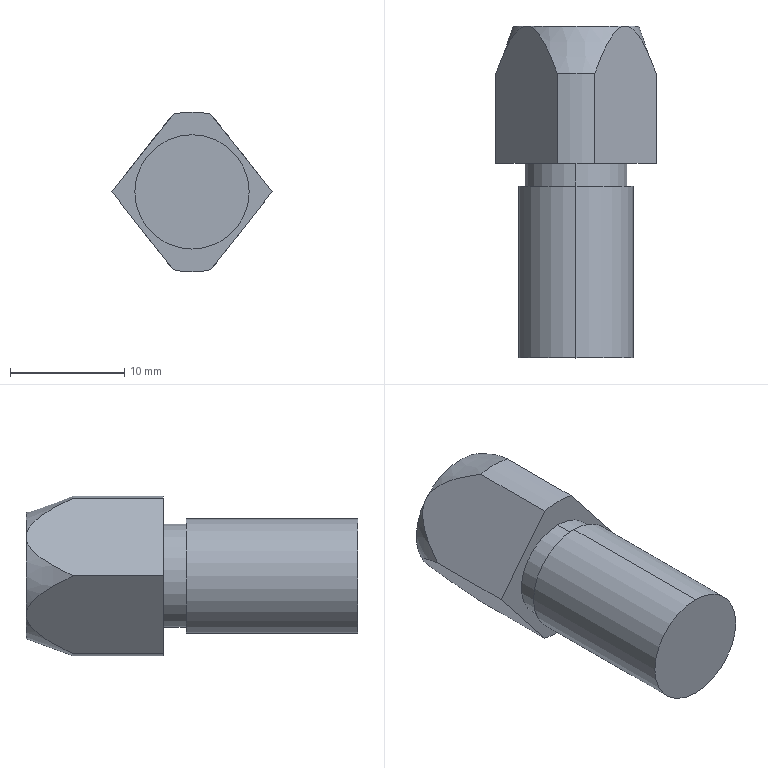Component | SolidWorks | 10-14DiamondPin-1 | 1 solid | 20 faces | box 14 x 29 x 14 mm | volume 2690 mm3 | plane 8 | cylinder 7 | cone 5 | commonest cylinder face diameters 14 x3 9 x2 10 x2
STEP:
#1=COLOUR_RGB('',0.7922,0.8196,0.9333);
#2=FILL_AREA_STYLE_COLOUR('',#1);
#3=FILL_AREA_STYLE('',(#2));
#4=SURFACE_STYLE_FILL_AREA(#3);
#5=SURFACE_SIDE_STYLE('',(#4));
#6=SURFACE_STYLE_USAGE(.BOTH.,#5);
#7=PRESENTATION_STYLE_ASSIGNMENT((#6));
#8=CARTESIAN_POINT('',(2.495,3.663,1.87));
#9=VERTEX_POINT('',#8);
#10=CARTESIAN_POINT('',(2.495,3.663,2.224));
#11=VERTEX_POINT('',#10);
#12=CARTESIAN_POINT('',(2.495,3.663,2.047));
#13=DIRECTION('',(0.,-1.,0.));
#14=DIRECTION('',(0.,0.,-1.));
#15=AXIS2_PLACEMENT_3D('',#12,#13,#14);
#16=CIRCLE('',#15,0.1772);
#17=EDGE_CURVE('',#9,#11,#16,.T.);
#18=ORIENTED_EDGE('',*,*,#17,.T.);
#19=CARTESIAN_POINT('',(2.495,3.585,2.224));
#20=VERTEX_POINT('',#19);
#21=CARTESIAN_POINT('',(2.495,2.994,2.224));
#22=DIRECTION('',(0.,-1.,0.));
#23=VECTOR('',#22,39.37);
#24=LINE('',#21,#23);
#25=EDGE_CURVE('',#11,#20,#24,.T.);
#26=ORIENTED_EDGE('',*,*,#25,.T.);
#27=CARTESIAN_POINT('',(2.495,3.585,1.87));
#28=VERTEX_POINT('',#27);
#29=CARTESIAN_POINT('',(2.495,3.585,2.047));
#30=DIRECTION('',(0.,-1.,0.));
#31=DIRECTION('',(0.,0.,-1.));
#32=AXIS2_PLACEMENT_3D('',#29,#30,#31);
#33=CIRCLE('',#32,0.1772);
#34=EDGE_CURVE('',#28,#20,#33,.T.);
#35=ORIENTED_EDGE('',*,*,#34,.F.);
#36=CARTESIAN_POINT('',(2.495,2.994,1.87));
#37=DIRECTION('',(0.,-1.,0.));
#38=VECTOR('',#37,39.37);
#39=LINE('',#36,#38);
#40=EDGE_CURVE('',#9,#28,#39,.T.);
#41=ORIENTED_EDGE('',*,*,#40,.F.);
#42=EDGE_LOOP('',(#18,#26,#35,#41));
#43=FACE_OUTER_BOUND('',#42,.T.);
#44=CARTESIAN_POINT('',(2.495,2.994,2.047));
#45=DIRECTION('',(0.,-1.,0.));
#46=DIRECTION('',(0.,0.,-1.));
#47=AXIS2_PLACEMENT_3D('',#44,#45,#46);
#48=CYLINDRICAL_SURFACE('',#47,0.1772);
#49=ADVANCED_FACE('',(#43),#48,.T.);
#50=CARTESIAN_POINT('',(2.495,3.585,1.85));
#51=VERTEX_POINT('',#50);
#52=CARTESIAN_POINT('',(2.495,3.585,2.244));
#53=VERTEX_POINT('',#52);
#54=CARTESIAN_POINT('',(2.495,3.585,2.047));
#55=DIRECTION('',(0.,-1.,0.));
#56=DIRECTION('',(0.,0.,-1.));
#57=AXIS2_PLACEMENT_3D('',#54,#55,#56);
#58=CIRCLE('',#57,0.1969);
#59=EDGE_CURVE('',#51,#53,#58,.T.);
#60=ORIENTED_EDGE('',*,*,#59,.T.);
#61=CARTESIAN_POINT('',(2.495,2.994,2.244));
#62=VERTEX_POINT('',#61);
#63=CARTESIAN_POINT('',(2.495,2.994,2.244));
#64=DIRECTION('',(0.,-1.,0.));
#65=VECTOR('',#64,39.37);
#66=LINE('',#63,#65);
#67=EDGE_CURVE('',#53,#62,#66,.T.);
#68=ORIENTED_EDGE('',*,*,#67,.T.);
#69=CARTESIAN_POINT('',(2.495,2.994,1.85));
#70=VERTEX_POINT('',#69);
#71=CARTESIAN_POINT('',(2.495,2.994,2.047));
#72=DIRECTION('',(0.,-1.,0.));
#73=DIRECTION('',(0.,0.,-1.));
#74=AXIS2_PLACEMENT_3D('',#71,#72,#73);
#75=CIRCLE('',#74,0.1969);
#76=EDGE_CURVE('',#70,#62,#75,.T.);
#77=ORIENTED_EDGE('',*,*,#76,.F.);
#78=CARTESIAN_POINT('',(2.495,2.994,1.85));
#79=DIRECTION('',(0.,-1.,0.));
#80=VECTOR('',#79,39.37);
#81=LINE('',#78,#80);
#82=EDGE_CURVE('',#51,#70,#81,.T.);
#83=ORIENTED_EDGE('',*,*,#82,.F.);
#84=EDGE_LOOP('',(#60,#68,#77,#83));
#85=FACE_OUTER_BOUND('',#84,.T.);
#86=CARTESIAN_POINT('',(2.495,2.994,2.047));
#87=DIRECTION('',(0.,-1.,0.));
#88=DIRECTION('',(0.,0.,-1.));
#89=AXIS2_PLACEMENT_3D('',#86,#87,#88);
#90=CYLINDRICAL_SURFACE('',#89,0.1969);
#91=ADVANCED_FACE('',(#85),#90,.T.);
#92=CARTESIAN_POINT('',(2.495,4.136,1.831));
#93=VERTEX_POINT('',#92);
#94=CARTESIAN_POINT('',(2.325,4.136,1.913));
#95=VERTEX_POINT('',#94);
#96=CARTESIAN_POINT('',(2.495,4.136,2.047));
#97=DIRECTION('',(0.,1.,0.));
#98=DIRECTION('',(0.,0.,1.));
#99=AXIS2_PLACEMENT_3D('',#96,#97,#98);
#100=CIRCLE('',#99,0.2165);
#101=EDGE_CURVE('',#93,#95,#100,.T.);
#102=ORIENTED_EDGE('',*,*,#101,.F.);
#103=CARTESIAN_POINT('',(2.495,3.973,1.772));
#104=VERTEX_POINT('',#103);
#105=CARTESIAN_POINT('',(2.495,3.973,1.772));
#106=DIRECTION('',(0.,-0.9397,-0.342));
#107=VECTOR('',#106,39.37);
#108=LINE('',#105,#107);
#109=EDGE_CURVE('',#93,#104,#108,.T.);
#110=ORIENTED_EDGE('',*,*,#109,.T.);
#111=CARTESIAN_POINT('',(2.431,3.973,1.779));
#112=VERTEX_POINT('',#111);
#113=CARTESIAN_POINT('',(2.495,3.973,2.047));
#114=DIRECTION('',(0.,-1.,0.));
#115=DIRECTION('',(0.,0.,1.));
#116=AXIS2_PLACEMENT_3D('',#113,#114,#115);
#117=CIRCLE('',#116,0.2756);
#118=EDGE_CURVE('',#112,#104,#117,.T.);
#119=ORIENTED_EDGE('',*,*,#118,.F.);
#120=CARTESIAN_POINT('',(2.325,4.136,1.913));
#121=CARTESIAN_POINT('',(2.328,4.136,1.909));
#122=CARTESIAN_POINT('',(2.331,4.135,1.905));
#123=CARTESIAN_POINT('',(2.338,4.133,1.897));
#124=CARTESIAN_POINT('',(2.341,4.132,1.894));
#125=CARTESIAN_POINT('',(2.35,4.126,1.882));
#126=CARTESIAN_POINT('',(2.355,4.121,1.875));
#127=CARTESIAN_POINT('',(2.366,4.11,1.862));
#128=CARTESIAN_POINT('',(2.37,4.103,1.856));
#129=CARTESIAN_POINT('',(2.379,4.089,1.844));
#130=CARTESIAN_POINT('',(2.384,4.082,1.839));
#131=CARTESIAN_POINT('',(2.396,4.058,1.823));
#132=CARTESIAN_POINT('',(2.404,4.042,1.814));
#133=CARTESIAN_POINT('',(2.418,4.008,1.796));
#134=CARTESIAN_POINT('',(2.424,3.991,1.787));
#135=CARTESIAN_POINT('',(2.431,3.973,1.779));
#136=B_SPLINE_CURVE_WITH_KNOTS('',3,(#120,#121,#122,#123,#124,#125,#126,#127,#128,#129,#130,#131,#132,#133,#134,#135),.UNSPECIFIED.,.F.,.F.,(4,2,2,2,2,2,2,4),(0.006199,0.006588,0.006976,0.007754,0.008531,0.009309,0.01086,0.01242),.UNSPECIFIED.);
#137=EDGE_CURVE('',#95,#112,#136,.T.);
#138=ORIENTED_EDGE('',*,*,#137,.F.);
#139=EDGE_LOOP('',(#102,#110,#119,#138));
#140=FACE_OUTER_BOUND('',#139,.T.);
#141=CARTESIAN_POINT('',(2.495,3.973,2.047));
#142=DIRECTION('',(0.,-1.,0.));
#143=DIRECTION('',(0.,0.,-1.));
#144=AXIS2_PLACEMENT_3D('',#141,#142,#143);
#145=CONICAL_SURFACE('',#144,0.2756,0.3491);
#146=ADVANCED_FACE('',(#140),#145,.T.);
#147=ORIENTED_EDGE('',*,*,#118,.T.);
#148=CARTESIAN_POINT('',(2.495,3.663,1.772));
#149=VERTEX_POINT('',#148);
#150=CARTESIAN_POINT('',(2.495,2.994,1.772));
#151=DIRECTION('',(0.,-1.,0.));
#152=VECTOR('',#151,39.37);
#153=LINE('',#150,#152);
#154=EDGE_CURVE('',#104,#149,#153,.T.);
#155=ORIENTED_EDGE('',*,*,#154,.T.);
#156=CARTESIAN_POINT('',(2.431,3.663,1.779));
#157=VERTEX_POINT('',#156);
#158=CARTESIAN_POINT('',(2.495,3.663,2.047));
#159=DIRECTION('',(0.,-1.,0.));
#160=DIRECTION('',(0.,0.,-1.));
#161=AXIS2_PLACEMENT_3D('',#158,#159,#160);
#162=CIRCLE('',#161,0.2756);
#163=EDGE_CURVE('',#157,#149,#162,.T.);
#164=ORIENTED_EDGE('',*,*,#163,.F.);
#165=CARTESIAN_POINT('',(2.431,3.348,1.779));
#166=DIRECTION('',(0.,1.,0.));
#167=VECTOR('',#166,39.37);
#168=LINE('',#165,#167);
#169=EDGE_CURVE('',#157,#112,#168,.T.);
#170=ORIENTED_EDGE('',*,*,#169,.T.);
#171=EDGE_LOOP('',(#147,#155,#164,#170));
#172=FACE_OUTER_BOUND('',#171,.T.);
#173=CARTESIAN_POINT('',(2.495,2.994,2.047));
#174=DIRECTION('',(0.,-1.,0.));
#175=DIRECTION('',(0.,0.,-1.));
#176=AXIS2_PLACEMENT_3D('',#173,#174,#175);
#177=CYLINDRICAL_SURFACE('',#176,0.2756);
#178=ADVANCED_FACE('',(#172),#177,.T.);
#179=CARTESIAN_POINT('',(2.22,3.973,2.047));
#180=VERTEX_POINT('',#179);
#181=CARTESIAN_POINT('',(2.22,3.973,2.047));
#182=CARTESIAN_POINT('',(2.226,3.991,2.039));
#183=CARTESIAN_POINT('',(2.233,4.008,2.031));
#184=CARTESIAN_POINT('',(2.247,4.042,2.013));
#185=CARTESIAN_POINT('',(2.254,4.058,2.003));
#186=CARTESIAN_POINT('',(2.267,4.082,1.988));
#187=CARTESIAN_POINT('',(2.271,4.089,1.982));
#188=CARTESIAN_POINT('',(2.28,4.103,1.971));
#189=CARTESIAN_POINT('',(2.285,4.11,1.964));
#190=CARTESIAN_POINT('',(2.295,4.121,1.951));
#191=CARTESIAN_POINT('',(2.301,4.126,1.944));
#192=CARTESIAN_POINT('',(2.31,4.132,1.933));
#193=CARTESIAN_POINT('',(2.313,4.133,1.929));
#194=CARTESIAN_POINT('',(2.319,4.135,1.921));
#195=CARTESIAN_POINT('',(2.322,4.136,1.917));
#196=CARTESIAN_POINT('',(2.325,4.136,1.913));
#197=B_SPLINE_CURVE_WITH_KNOTS('',3,(#181,#182,#183,#184,#185,#186,#187,#188,#189,#190,#191,#192,#193,#194,#195,#196),.UNSPECIFIED.,.F.,.F.,(4,2,2,2,2,2,2,4),(0.00000023,0.00155,0.0031,0.003875,0.004649,0.005424,0.005812,0.006199),.UNSPECIFIED.);
#198=EDGE_CURVE('',#180,#95,#197,.T.);
#199=ORIENTED_EDGE('',*,*,#198,.F.);
#200=CARTESIAN_POINT('',(2.325,4.136,2.181));
#201=VERTEX_POINT('',#200);
#202=CARTESIAN_POINT('',(2.22,3.973,2.047));
#203=CARTESIAN_POINT('',(2.226,3.991,2.055));
#204=CARTESIAN_POINT('',(2.233,4.008,2.064));
#205=CARTESIAN_POINT('',(2.247,4.042,2.082));
#206=CARTESIAN_POINT('',(2.254,4.058,2.091));
#207=CARTESIAN_POINT('',(2.267,4.082,2.107));
#208=CARTESIAN_POINT('',(2.271,4.089,2.112));
#209=CARTESIAN_POINT('',(2.28,4.103,2.124));
#210=CARTESIAN_POINT('',(2.285,4.11,2.13));
#211=CARTESIAN_POINT('',(2.295,4.121,2.143));
#212=CARTESIAN_POINT('',(2.301,4.126,2.15));
#213=CARTESIAN_POINT('',(2.31,4.132,2.161));
#214=CARTESIAN_POINT('',(2.313,4.133,2.165));
#215=CARTESIAN_POINT('',(2.319,4.135,2.173));
#216=CARTESIAN_POINT('',(2.322,4.136,2.177));
#217=CARTESIAN_POINT('',(2.325,4.136,2.181));
#218=B_SPLINE_CURVE_WITH_KNOTS('',3,(#202,#203,#204,#205,#206,#207,#208,#209,#210,#211,#212,#213,#214,#215,#216,#217),.UNSPECIFIED.,.F.,.F.,(4,2,2,2,2,2,2,4),(0.00000023,0.00155,0.0031,0.003875,0.004649,0.005424,0.005812,0.006199),.UNSPECIFIED.);
#219=EDGE_CURVE('',#180,#201,#218,.T.);
#220=ORIENTED_EDGE('',*,*,#219,.T.);
#221=CARTESIAN_POINT('',(2.495,4.136,2.047));
#222=DIRECTION('',(0.,1.,0.));
#223=DIRECTION('',(0.,0.,1.));
#224=AXIS2_PLACEMENT_3D('',#221,#222,#223);
#225=CIRCLE('',#224,0.2165);
#226=EDGE_CURVE('',#95,#201,#225,.T.);
#227=ORIENTED_EDGE('',*,*,#226,.F.);
#228=EDGE_LOOP('',(#199,#220,#227));
#229=FACE_OUTER_BOUND('',#228,.T.);
#230=CARTESIAN_POINT('',(2.495,3.973,2.047));
#231=DIRECTION('',(0.,-1.,0.));
#232=DIRECTION('',(0.,0.,-1.));
#233=AXIS2_PLACEMENT_3D('',#230,#231,#232);
#234=CONICAL_SURFACE('',#233,0.2756,0.3491);
#235=ADVANCED_FACE('',(#229),#234,.T.);
#236=CARTESIAN_POINT('',(2.771,3.973,2.047));
#237=VERTEX_POINT('',#236);
#238=CARTESIAN_POINT('',(2.665,4.136,2.181));
#239=VERTEX_POINT('',#238);
#240=CARTESIAN_POINT('',(2.771,3.973,2.047));
#241=CARTESIAN_POINT('',(2.765,3.991,2.055));
#242=CARTESIAN_POINT('',(2.758,4.008,2.064));
#243=CARTESIAN_POINT('',(2.744,4.042,2.082));
#244=CARTESIAN_POINT('',(2.736,4.058,2.091));
#245=CARTESIAN_POINT('',(2.724,4.082,2.107));
#246=CARTESIAN_POINT('',(2.72,4.089,2.112));
#247=CARTESIAN_POINT('',(2.711,4.103,2.124));
#248=CARTESIAN_POINT('',(2.706,4.11,2.13));
#249=CARTESIAN_POINT('',(2.695,4.121,2.143));
#250=CARTESIAN_POINT('',(2.69,4.126,2.15));
#251=CARTESIAN_POINT('',(2.681,4.132,2.161));
#252=CARTESIAN_POINT('',(2.678,4.133,2.165));
#253=CARTESIAN_POINT('',(2.672,4.135,2.173));
#254=CARTESIAN_POINT('',(2.669,4.136,2.177));
#255=CARTESIAN_POINT('',(2.665,4.136,2.181));
#256=B_SPLINE_CURVE_WITH_KNOTS('',3,(#240,#241,#242,#243,#244,#245,#246,#247,#248,#249,#250,#251,#252,#253,#254,#255),.UNSPECIFIED.,.F.,.F.,(4,2,2,2,2,2,2,4),(0.00000023,0.00155,0.0031,0.003875,0.004649,0.005424,0.005812,0.006199),.UNSPECIFIED.);
#257=EDGE_CURVE('',#237,#239,#256,.T.);
#258=ORIENTED_EDGE('',*,*,#257,.F.);
#259=CARTESIAN_POINT('',(2.665,4.136,1.913));
#260=VERTEX_POINT('',#259);
#261=CARTESIAN_POINT('',(2.771,3.973,2.047));
#262=CARTESIAN_POINT('',(2.765,3.991,2.039));
#263=CARTESIAN_POINT('',(2.758,4.008,2.031));
#264=CARTESIAN_POINT('',(2.744,4.042,2.013));
#265=CARTESIAN_POINT('',(2.736,4.058,2.003));
#266=CARTESIAN_POINT('',(2.724,4.082,1.988));
#267=CARTESIAN_POINT('',(2.72,4.089,1.982));
#268=CARTESIAN_POINT('',(2.711,4.103,1.971));
#269=CARTESIAN_POINT('',(2.706,4.11,1.964));
#270=CARTESIAN_POINT('',(2.695,4.121,1.951));
#271=CARTESIAN_POINT('',(2.69,4.126,1.944));
#272=CARTESIAN_POINT('',(2.681,4.132,1.933));
#273=CARTESIAN_POINT('',(2.678,4.133,1.929));
#274=CARTESIAN_POINT('',(2.672,4.135,1.921));
#275=CARTESIAN_POINT('',(2.669,4.136,1.917));
#276=CARTESIAN_POINT('',(2.665,4.136,1.913));
#277=B_SPLINE_CURVE_WITH_KNOTS('',3,(#261,#262,#263,#264,#265,#266,#267,#268,#269,#270,#271,#272,#273,#274,#275,#276),.UNSPECIFIED.,.F.,.F.,(4,2,2,2,2,2,2,4),(0.00000023,0.00155,0.0031,0.003875,0.004649,0.005424,0.005812,0.006199),.UNSPECIFIED.);
#278=EDGE_CURVE('',#237,#260,#277,.T.);
#279=ORIENTED_EDGE('',*,*,#278,.T.);
#280=CARTESIAN_POINT('',(2.495,4.136,2.047));
#281=DIRECTION('',(0.,1.,0.));
#282=DIRECTION('',(0.,0.,1.));
#283=AXIS2_PLACEMENT_3D('',#280,#281,#282);
#284=CIRCLE('',#283,0.2165);
#285=EDGE_CURVE('',#239,#260,#284,.T.);
#286=ORIENTED_EDGE('',*,*,#285,.F.);
#287=EDGE_LOOP('',(#258,#279,#286));
#288=FACE_OUTER_BOUND('',#287,.T.);
#289=CARTESIAN_POINT('',(2.495,3.973,2.047));
#290=DIRECTION('',(0.,-1.,0.));
#291=DIRECTION('',(0.,0.,-1.));
#292=AXIS2_PLACEMENT_3D('',#289,#290,#291);
#293=CONICAL_SURFACE('',#292,0.2756,0.3491);
#294=ADVANCED_FACE('',(#288),#293,.T.);
#295=CARTESIAN_POINT('',(2.22,3.663,2.047));
#296=VERTEX_POINT('',#295);
#297=CARTESIAN_POINT('',(2.411,3.663,1.804));
#298=DIRECTION('',(-0.6186,0.,0.7857));
#299=VECTOR('',#298,39.37);
#300=LINE('',#297,#299);
#301=EDGE_CURVE('',#157,#296,#300,.T.);
#302=ORIENTED_EDGE('',*,*,#301,.F.);
#303=ORIENTED_EDGE('',*,*,#163,.T.);
#304=CARTESIAN_POINT('',(2.56,3.663,1.779));
#305=VERTEX_POINT('',#304);
#306=CARTESIAN_POINT('',(2.495,3.663,2.047));
#307=DIRECTION('',(0.,-1.,0.));
#308=DIRECTION('',(0.,0.,-1.));
#309=AXIS2_PLACEMENT_3D('',#306,#307,#308);
#310=CIRCLE('',#309,0.2756);
#311=EDGE_CURVE('',#149,#305,#310,.T.);
#312=ORIENTED_EDGE('',*,*,#311,.T.);
#313=CARTESIAN_POINT('',(2.771,3.663,2.047));
#314=VERTEX_POINT('',#313);
#315=CARTESIAN_POINT('',(2.579,3.663,1.804));
#316=DIRECTION('',(0.6186,0.,0.7857));
#317=VECTOR('',#316,39.37);
#318=LINE('',#315,#317);
#319=EDGE_CURVE('',#305,#314,#318,.T.);
#320=ORIENTED_EDGE('',*,*,#319,.T.);
#321=CARTESIAN_POINT('',(2.56,3.663,2.315));
#322=VERTEX_POINT('',#321);
#323=CARTESIAN_POINT('',(2.752,3.663,2.072));
#324=DIRECTION('',(0.6186,0.,-0.7857));
#325=VECTOR('',#324,39.37);
#326=LINE('',#323,#325);
#327=EDGE_CURVE('',#322,#314,#326,.T.);
#328=ORIENTED_EDGE('',*,*,#327,.F.);
#329=CARTESIAN_POINT('',(2.431,3.663,2.315));
#330=VERTEX_POINT('',#329);
#331=CARTESIAN_POINT('',(2.495,3.663,2.047));
#332=DIRECTION('',(0.,-1.,0.));
#333=DIRECTION('',(0.,0.,-1.));
#334=AXIS2_PLACEMENT_3D('',#331,#332,#333);
#335=CIRCLE('',#334,0.2756);
#336=EDGE_CURVE('',#322,#330,#335,.T.);
#337=ORIENTED_EDGE('',*,*,#336,.T.);
#338=CARTESIAN_POINT('',(2.239,3.663,2.072));
#339=DIRECTION('',(-0.6186,0.,-0.7857));
#340=VECTOR('',#339,39.37);
#341=LINE('',#338,#340);
#342=EDGE_CURVE('',#330,#296,#341,.T.);
#343=ORIENTED_EDGE('',*,*,#342,.T.);
#344=EDGE_LOOP('',(#302,#303,#312,#320,#328,#337,#343));
#345=FACE_OUTER_BOUND('',#344,.T.);
#346=ORIENTED_EDGE('',*,*,#17,.F.);
#347=CARTESIAN_POINT('',(2.495,3.663,2.047));
#348=DIRECTION('',(0.,-1.,0.));
#349=DIRECTION('',(0.,0.,-1.));
#350=AXIS2_PLACEMENT_3D('',#347,#348,#349);
#351=CIRCLE('',#350,0.1772);
#352=EDGE_CURVE('',#11,#9,#351,.T.);
#353=ORIENTED_EDGE('',*,*,#352,.F.);
#354=EDGE_LOOP('',(#346,#353));
#355=FACE_BOUND('',#354,.T.);
#356=CARTESIAN_POINT('',(2.495,3.663,1.87));
#357=DIRECTION('',(0.,-1.,0.));
#358=DIRECTION('',(0.,0.,-1.));
#359=AXIS2_PLACEMENT_3D('',#356,#357,#358);
#360=PLANE('',#359);
#361=ADVANCED_FACE('',(#345,#355),#360,.T.);
#362=ORIENTED_EDGE('',*,*,#154,.F.);
#363=CARTESIAN_POINT('',(2.56,3.973,1.779));
#364=VERTEX_POINT('',#363);
#365=CARTESIAN_POINT('',(2.495,3.973,2.047));
#366=DIRECTION('',(0.,-1.,0.));
#367=DIRECTION('',(0.,0.,1.));
#368=AXIS2_PLACEMENT_3D('',#365,#366,#367);
#369=CIRCLE('',#368,0.2756);
#370=EDGE_CURVE('',#104,#364,#369,.T.);
#371=ORIENTED_EDGE('',*,*,#370,.T.);
#372=CARTESIAN_POINT('',(2.56,3.348,1.779));
#373=DIRECTION('',(0.,1.,0.));
#374=VECTOR('',#373,39.37);
#375=LINE('',#372,#374);
#376=EDGE_CURVE('',#305,#364,#375,.T.);
#377=ORIENTED_EDGE('',*,*,#376,.F.);
#378=ORIENTED_EDGE('',*,*,#311,.F.);
#379=EDGE_LOOP('',(#362,#371,#377,#378));
#380=FACE_OUTER_BOUND('',#379,.T.);
#381=CARTESIAN_POINT('',(2.495,2.994,2.047));
#382=DIRECTION('',(0.,-1.,0.));
#383=DIRECTION('',(0.,0.,-1.));
#384=AXIS2_PLACEMENT_3D('',#381,#382,#383);
#385=CYLINDRICAL_SURFACE('',#384,0.2756);
#386=ADVANCED_FACE('',(#380),#385,.T.);
#387=CARTESIAN_POINT('',(2.56,3.973,2.315));
#388=VERTEX_POINT('',#387);
#389=CARTESIAN_POINT('',(2.56,3.348,2.315));
#390=DIRECTION('',(0.,1.,0.));
#391=VECTOR('',#390,39.37);
#392=LINE('',#389,#391);
#393=EDGE_CURVE('',#322,#388,#392,.T.);
#394=ORIENTED_EDGE('',*,*,#393,.T.);
#395=CARTESIAN_POINT('',(2.431,3.973,2.315));
#396=VERTEX_POINT('',#395);
#397=CARTESIAN_POINT('',(2.495,3.973,2.047));
#398=DIRECTION('',(0.,-1.,0.));
#399=DIRECTION('',(0.,0.,1.));
#400=AXIS2_PLACEMENT_3D('',#397,#398,#399);
#401=CIRCLE('',#400,0.2756);
#402=EDGE_CURVE('',#388,#396,#401,.T.);
#403=ORIENTED_EDGE('',*,*,#402,.T.);
#404=CARTESIAN_POINT('',(2.431,3.348,2.315));
#405=DIRECTION('',(0.,1.,0.));
#406=VECTOR('',#405,39.37);
#407=LINE('',#404,#406);
#408=EDGE_CURVE('',#330,#396,#407,.T.);
#409=ORIENTED_EDGE('',*,*,#408,.F.);
#410=ORIENTED_EDGE('',*,*,#336,.F.);
#411=EDGE_LOOP('',(#394,#403,#409,#410));
#412=FACE_OUTER_BOUND('',#411,.T.);
#413=CARTESIAN_POINT('',(2.495,2.994,2.047));
#414=DIRECTION('',(0.,-1.,0.));
#415=DIRECTION('',(0.,0.,-1.));
#416=AXIS2_PLACEMENT_3D('',#413,#414,#415);
#417=CYLINDRICAL_SURFACE('',#416,0.2756);
#418=ADVANCED_FACE('',(#412),#417,.T.);
#419=ORIENTED_EDGE('',*,*,#109,.F.);
#420=CARTESIAN_POINT('',(2.495,4.136,2.047));
#421=DIRECTION('',(0.,1.,0.));
#422=DIRECTION('',(0.,0.,1.));
#423=AXIS2_PLACEMENT_3D('',#420,#421,#422);
#424=CIRCLE('',#423,0.2165);
#425=EDGE_CURVE('',#260,#93,#424,.T.);
#426=ORIENTED_EDGE('',*,*,#425,.F.);
#427=CARTESIAN_POINT('',(2.665,4.136,1.913));
#428=CARTESIAN_POINT('',(2.662,4.136,1.909));
#429=CARTESIAN_POINT('',(2.659,4.135,1.905));
#430=CARTESIAN_POINT('',(2.653,4.133,1.897));
#431=CARTESIAN_POINT('',(2.65,4.132,1.894));
#432=CARTESIAN_POINT('',(2.641,4.126,1.882));
#433=CARTESIAN_POINT('',(2.636,4.121,1.875));
#434=CARTESIAN_POINT('',(2.625,4.11,1.862));
#435=CARTESIAN_POINT('',(2.62,4.103,1.856));
#436=CARTESIAN_POINT('',(2.611,4.089,1.844));
#437=CARTESIAN_POINT('',(2.607,4.082,1.839));
#438=CARTESIAN_POINT('',(2.595,4.058,1.823));
#439=CARTESIAN_POINT('',(2.587,4.042,1.814));
#440=CARTESIAN_POINT('',(2.573,4.008,1.796));
#441=CARTESIAN_POINT('',(2.566,3.991,1.787));
#442=CARTESIAN_POINT('',(2.56,3.973,1.779));
#443=B_SPLINE_CURVE_WITH_KNOTS('',3,(#427,#428,#429,#430,#431,#432,#433,#434,#435,#436,#437,#438,#439,#440,#441,#442),.UNSPECIFIED.,.F.,.F.,(4,2,2,2,2,2,2,4),(0.006199,0.006588,0.006976,0.007754,0.008531,0.009309,0.01086,0.01242),.UNSPECIFIED.);
#444=EDGE_CURVE('',#260,#364,#443,.T.);
#445=ORIENTED_EDGE('',*,*,#444,.T.);
#446=ORIENTED_EDGE('',*,*,#370,.F.);
#447=EDGE_LOOP('',(#419,#426,#445,#446));
#448=FACE_OUTER_BOUND('',#447,.T.);
#449=CARTESIAN_POINT('',(2.495,3.973,2.047));
#450=DIRECTION('',(0.,-1.,0.));
#451=DIRECTION('',(0.,0.,-1.));
#452=AXIS2_PLACEMENT_3D('',#449,#450,#451);
#453=CONICAL_SURFACE('',#452,0.2756,0.3491);
#454=ADVANCED_FACE('',(#448),#453,.T.);
#455=CARTESIAN_POINT('',(2.665,4.136,2.181));
#456=CARTESIAN_POINT('',(2.662,4.136,2.185));
#457=CARTESIAN_POINT('',(2.659,4.135,2.189));
#458=CARTESIAN_POINT('',(2.653,4.133,2.197));
#459=CARTESIAN_POINT('',(2.65,4.132,2.201));
#460=CARTESIAN_POINT('',(2.641,4.126,2.212));
#461=CARTESIAN_POINT('',(2.636,4.121,2.219));
#462=CARTESIAN_POINT('',(2.625,4.11,2.232));
#463=CARTESIAN_POINT('',(2.62,4.103,2.239));
#464=CARTESIAN_POINT('',(2.611,4.089,2.25));
#465=CARTESIAN_POINT('',(2.607,4.082,2.256));
#466=CARTESIAN_POINT('',(2.595,4.058,2.271));
#467=CARTESIAN_POINT('',(2.587,4.042,2.281));
#468=CARTESIAN_POINT('',(2.573,4.008,2.299));
#469=CARTESIAN_POINT('',(2.566,3.991,2.307));
#470=CARTESIAN_POINT('',(2.56,3.973,2.315));
#471=B_SPLINE_CURVE_WITH_KNOTS('',3,(#455,#456,#457,#458,#459,#460,#461,#462,#463,#464,#465,#466,#467,#468,#469,#470),.UNSPECIFIED.,.F.,.F.,(4,2,2,2,2,2,2,4),(0.006199,0.006588,0.006976,0.007754,0.008531,0.009309,0.01086,0.01242),.UNSPECIFIED.);
#472=EDGE_CURVE('',#239,#388,#471,.T.);
#473=ORIENTED_EDGE('',*,*,#472,.F.);
#474=CARTESIAN_POINT('',(2.495,4.136,2.047));
#475=DIRECTION('',(0.,1.,0.));
#476=DIRECTION('',(0.,0.,1.));
#477=AXIS2_PLACEMENT_3D('',#474,#475,#476);
#478=CIRCLE('',#477,0.2165);
#479=EDGE_CURVE('',#201,#239,#478,.T.);
#480=ORIENTED_EDGE('',*,*,#479,.F.);
#481=CARTESIAN_POINT('',(2.325,4.136,2.181));
#482=CARTESIAN_POINT('',(2.328,4.136,2.185));
#483=CARTESIAN_POINT('',(2.331,4.135,2.189));
#484=CARTESIAN_POINT('',(2.338,4.133,2.197));
#485=CARTESIAN_POINT('',(2.341,4.132,2.201));
#486=CARTESIAN_POINT('',(2.35,4.126,2.212));
#487=CARTESIAN_POINT('',(2.355,4.121,2.219));
#488=CARTESIAN_POINT('',(2.366,4.11,2.232));
#489=CARTESIAN_POINT('',(2.37,4.103,2.239));
#490=CARTESIAN_POINT('',(2.379,4.089,2.25));
#491=CARTESIAN_POINT('',(2.384,4.082,2.256));
#492=CARTESIAN_POINT('',(2.396,4.058,2.271));
#493=CARTESIAN_POINT('',(2.404,4.042,2.281));
#494=CARTESIAN_POINT('',(2.418,4.008,2.299));
#495=CARTESIAN_POINT('',(2.424,3.991,2.307));
#496=CARTESIAN_POINT('',(2.431,3.973,2.315));
#497=B_SPLINE_CURVE_WITH_KNOTS('',3,(#481,#482,#483,#484,#485,#486,#487,#488,#489,#490,#491,#492,#493,#494,#495,#496),.UNSPECIFIED.,.F.,.F.,(4,2,2,2,2,2,2,4),(0.006199,0.006588,0.006976,0.007754,0.008531,0.009309,0.01086,0.01242),.UNSPECIFIED.);
#498=EDGE_CURVE('',#201,#396,#497,.T.);
#499=ORIENTED_EDGE('',*,*,#498,.T.);
#500=ORIENTED_EDGE('',*,*,#402,.F.);
#501=EDGE_LOOP('',(#473,#480,#499,#500));
#502=FACE_OUTER_BOUND('',#501,.T.);
#503=CARTESIAN_POINT('',(2.495,3.973,2.047));
#504=DIRECTION('',(0.,-1.,0.));
#505=DIRECTION('',(0.,0.,-1.));
#506=AXIS2_PLACEMENT_3D('',#503,#504,#505);
#507=CONICAL_SURFACE('',#506,0.2756,0.3491);
#508=ADVANCED_FACE('',(#502),#507,.T.);
#509=ORIENTED_EDGE('',*,*,#76,.T.);
#510=CARTESIAN_POINT('',(2.495,2.994,2.047));
#511=DIRECTION('',(0.,-1.,0.));
#512=DIRECTION('',(0.,0.,-1.));
#513=AXIS2_PLACEMENT_3D('',#510,#511,#512);
#514=CIRCLE('',#513,0.1969);
#515=EDGE_CURVE('',#62,#70,#514,.T.);
#516=ORIENTED_EDGE('',*,*,#515,.T.);
#517=EDGE_LOOP('',(#509,#516));
#518=FACE_OUTER_BOUND('',#517,.T.);
#519=CARTESIAN_POINT('',(2.495,2.994,2.047));
#520=DIRECTION('',(0.,-1.,0.));
#521=DIRECTION('',(0.,0.,-1.));
#522=AXIS2_PLACEMENT_3D('',#519,#520,#521);
#523=PLANE('',#522);
#524=ADVANCED_FACE('',(#518),#523,.T.);
#525=ORIENTED_EDGE('',*,*,#67,.F.);
#526=CARTESIAN_POINT('',(2.495,3.585,2.047));
#527=DIRECTION('',(0.,-1.,0.));
#528=DIRECTION('',(0.,0.,-1.));
#529=AXIS2_PLACEMENT_3D('',#526,#527,#528);
#530=CIRCLE('',#529,0.1969);
#531=EDGE_CURVE('',#53,#51,#530,.T.);
#532=ORIENTED_EDGE('',*,*,#531,.T.);
#533=ORIENTED_EDGE('',*,*,#82,.T.);
#534=ORIENTED_EDGE('',*,*,#515,.F.);
#535=EDGE_LOOP('',(#525,#532,#533,#534));
#536=FACE_OUTER_BOUND('',#535,.T.);
#537=CARTESIAN_POINT('',(2.495,2.994,2.047));
#538=DIRECTION('',(0.,-1.,0.));
#539=DIRECTION('',(0.,0.,-1.));
#540=AXIS2_PLACEMENT_3D('',#537,#538,#539);
#541=CYLINDRICAL_SURFACE('',#540,0.1969);
#542=ADVANCED_FACE('',(#536),#541,.T.);
#543=ORIENTED_EDGE('',*,*,#34,.T.);
#544=CARTESIAN_POINT('',(2.495,3.585,2.047));
#545=DIRECTION('',(0.,-1.,0.));
#546=DIRECTION('',(0.,0.,-1.));
#547=AXIS2_PLACEMENT_3D('',#544,#545,#546);
#548=CIRCLE('',#547,0.1772);
#549=EDGE_CURVE('',#20,#28,#548,.T.);
#550=ORIENTED_EDGE('',*,*,#549,.T.);
#551=EDGE_LOOP('',(#543,#550));
#552=FACE_BOUND('',#551,.T.);
#553=ORIENTED_EDGE('',*,*,#59,.F.);
#554=ORIENTED_EDGE('',*,*,#531,.F.);
#555=EDGE_LOOP('',(#553,#554));
#556=FACE_OUTER_BOUND('',#555,.T.);
#557=CARTESIAN_POINT('',(2.495,3.585,1.85));
#558=DIRECTION('',(0.,1.,0.));
#559=DIRECTION('',(0.,0.,1.));
#560=AXIS2_PLACEMENT_3D('',#557,#558,#559);
#561=PLANE('',#560);
#562=ADVANCED_FACE('',(#552,#556),#561,.T.);
#563=ORIENTED_EDGE('',*,*,#25,.F.);
#564=ORIENTED_EDGE('',*,*,#352,.T.);
#565=ORIENTED_EDGE('',*,*,#40,.T.);
#566=ORIENTED_EDGE('',*,*,#549,.F.);
#567=EDGE_LOOP('',(#563,#564,#565,#566));
#568=FACE_OUTER_BOUND('',#567,.T.);
#569=CARTESIAN_POINT('',(2.495,2.994,2.047));
#570=DIRECTION('',(0.,-1.,0.));
#571=DIRECTION('',(0.,0.,-1.));
#572=AXIS2_PLACEMENT_3D('',#569,#570,#571);
#573=CYLINDRICAL_SURFACE('',#572,0.1772);
#574=ADVANCED_FACE('',(#568),#573,.T.);
#575=ORIENTED_EDGE('',*,*,#425,.T.);
#576=ORIENTED_EDGE('',*,*,#101,.T.);
#577=ORIENTED_EDGE('',*,*,#226,.T.);
#578=ORIENTED_EDGE('',*,*,#479,.T.);
#579=ORIENTED_EDGE('',*,*,#285,.T.);
#580=EDGE_LOOP('',(#575,#576,#577,#578,#579));
#581=FACE_OUTER_BOUND('',#580,.T.);
#582=CARTESIAN_POINT('',(2.495,4.136,1.772));
#583=DIRECTION('',(0.,1.,0.));
#584=DIRECTION('',(0.,0.,1.));
#585=AXIS2_PLACEMENT_3D('',#582,#583,#584);
#586=PLANE('',#585);
#587=ADVANCED_FACE('',(#581),#586,.T.);
#588=ORIENTED_EDGE('',*,*,#376,.T.);
#589=ORIENTED_EDGE('',*,*,#444,.F.);
#590=ORIENTED_EDGE('',*,*,#278,.F.);
#591=CARTESIAN_POINT('',(2.771,3.348,2.047));
#592=DIRECTION('',(0.,1.,0.));
#593=VECTOR('',#592,39.37);
#594=LINE('',#591,#593);
#595=EDGE_CURVE('',#314,#237,#594,.T.);
#596=ORIENTED_EDGE('',*,*,#595,.F.);
#597=ORIENTED_EDGE('',*,*,#319,.F.);
#598=EDGE_LOOP('',(#588,#589,#590,#596,#597));
#599=FACE_OUTER_BOUND('',#598,.T.);
#600=CARTESIAN_POINT('',(2.665,3.348,1.913));
#601=DIRECTION('',(0.7857,0.,-0.6186));
#602=DIRECTION('',(-0.6186,0.,-0.7857));
#603=AXIS2_PLACEMENT_3D('',#600,#601,#602);
#604=PLANE('',#603);
#605=ADVANCED_FACE('',(#599),#604,.T.);
#606=ORIENTED_EDGE('',*,*,#408,.T.);
#607=ORIENTED_EDGE('',*,*,#498,.F.);
#608=ORIENTED_EDGE('',*,*,#219,.F.);
#609=CARTESIAN_POINT('',(2.22,3.348,2.047));
#610=DIRECTION('',(0.,1.,0.));
#611=VECTOR('',#610,39.37);
#612=LINE('',#609,#611);
#613=EDGE_CURVE('',#296,#180,#612,.T.);
#614=ORIENTED_EDGE('',*,*,#613,.F.);
#615=ORIENTED_EDGE('',*,*,#342,.F.);
#616=EDGE_LOOP('',(#606,#607,#608,#614,#615));
#617=FACE_OUTER_BOUND('',#616,.T.);
#618=CARTESIAN_POINT('',(2.325,3.348,2.181));
#619=DIRECTION('',(-0.7857,0.,0.6186));
#620=DIRECTION('',(0.6186,0.,0.7857));
#621=AXIS2_PLACEMENT_3D('',#618,#619,#620);
#622=PLANE('',#621);
#623=ADVANCED_FACE('',(#617),#622,.T.);
#624=ORIENTED_EDGE('',*,*,#301,.T.);
#625=ORIENTED_EDGE('',*,*,#613,.T.);
#626=ORIENTED_EDGE('',*,*,#198,.T.);
#627=ORIENTED_EDGE('',*,*,#137,.T.);
#628=ORIENTED_EDGE('',*,*,#169,.F.);
#629=EDGE_LOOP('',(#624,#625,#626,#627,#628));
#630=FACE_OUTER_BOUND('',#629,.T.);
#631=CARTESIAN_POINT('',(2.325,3.348,1.913));
#632=DIRECTION('',(0.7857,0.,0.6186));
#633=DIRECTION('',(0.6186,0.,-0.7857));
#634=AXIS2_PLACEMENT_3D('',#631,#632,#633);
#635=PLANE('',#634);
#636=ADVANCED_FACE('',(#630),#635,.F.);
#637=ORIENTED_EDGE('',*,*,#327,.T.);
#638=ORIENTED_EDGE('',*,*,#595,.T.);
#639=ORIENTED_EDGE('',*,*,#257,.T.);
#640=ORIENTED_EDGE('',*,*,#472,.T.);
#641=ORIENTED_EDGE('',*,*,#393,.F.);
#642=EDGE_LOOP('',(#637,#638,#639,#640,#641));
#643=FACE_OUTER_BOUND('',#642,.T.);
#644=CARTESIAN_POINT('',(2.665,3.348,2.181));
#645=DIRECTION('',(-0.7857,0.,-0.6186));
#646=DIRECTION('',(-0.6186,0.,0.7857));
#647=AXIS2_PLACEMENT_3D('',#644,#645,#646);
#648=PLANE('',#647);
#649=ADVANCED_FACE('',(#643),#648,.F.);
#650=CLOSED_SHELL('',(#49,#91,#146,#178,#235,#294,#361,#386,#418,#454,#508,#524,#542,#562,#574,#587,#605,#623,#636,#649));
#651=MANIFOLD_SOLID_BREP('',#650);
#652=STYLED_ITEM('',(#7),#651);
#653=(LENGTH_UNIT()NAMED_UNIT(*)SI_UNIT($,.METRE.));
#654=LENGTH_MEASURE_WITH_UNIT(LENGTH_MEASURE(0.0254),#653);
#655=DIMENSIONAL_EXPONENTS(1.,0.,0.,0.,0.,0.,0.);
#656=(CONVERSION_BASED_UNIT('',#654)LENGTH_UNIT()NAMED_UNIT(#655));
#657=UNCERTAINTY_MEASURE_WITH_UNIT(LENGTH_MEASURE(0.00001),#656,'','');
#658=(NAMED_UNIT(*)PLANE_ANGLE_UNIT()SI_UNIT($,.RADIAN.));
#659=(NAMED_UNIT(*)SI_UNIT($,.STERADIAN.)SOLID_ANGLE_UNIT());
#660=(GEOMETRIC_REPRESENTATION_CONTEXT(3)GLOBAL_UNCERTAINTY_ASSIGNED_CONTEXT((#657))GLOBAL_UNIT_ASSIGNED_CONTEXT((#656,#658,#659))REPRESENTATION_CONTEXT('',''));
#661=MECHANICAL_DESIGN_GEOMETRIC_PRESENTATION_REPRESENTATION('',(#652),#660);
#662=CARTESIAN_POINT('',(0.,0.,0.));
#663=DIRECTION('',(0.,0.,1.));
#664=DIRECTION('',(1.,0.,0.));
#665=AXIS2_PLACEMENT_3D('',#662,#663,#664);
#666=(LENGTH_UNIT()NAMED_UNIT(*)SI_UNIT($,.METRE.));
#667=LENGTH_MEASURE_WITH_UNIT(LENGTH_MEASURE(0.0254),#666);
#668=DIMENSIONAL_EXPONENTS(1.,0.,0.,0.,0.,0.,0.);
#669=(CONVERSION_BASED_UNIT('',#667)LENGTH_UNIT()NAMED_UNIT(#668));
#670=UNCERTAINTY_MEASURE_WITH_UNIT(LENGTH_MEASURE(0.00001),#669,'','');
#671=(NAMED_UNIT(*)PLANE_ANGLE_UNIT()SI_UNIT($,.RADIAN.));
#672=(NAMED_UNIT(*)SI_UNIT($,.STERADIAN.)SOLID_ANGLE_UNIT());
#673=(GEOMETRIC_REPRESENTATION_CONTEXT(3)GLOBAL_UNCERTAINTY_ASSIGNED_CONTEXT((#670))GLOBAL_UNIT_ASSIGNED_CONTEXT((#669,#671,#672))REPRESENTATION_CONTEXT('',''));
#674=ADVANCED_BREP_SHAPE_REPRESENTATION('',(#651,#665),#673);
#675=PRESENTATION_LAYER_ASSIGNMENT('','',(#652));